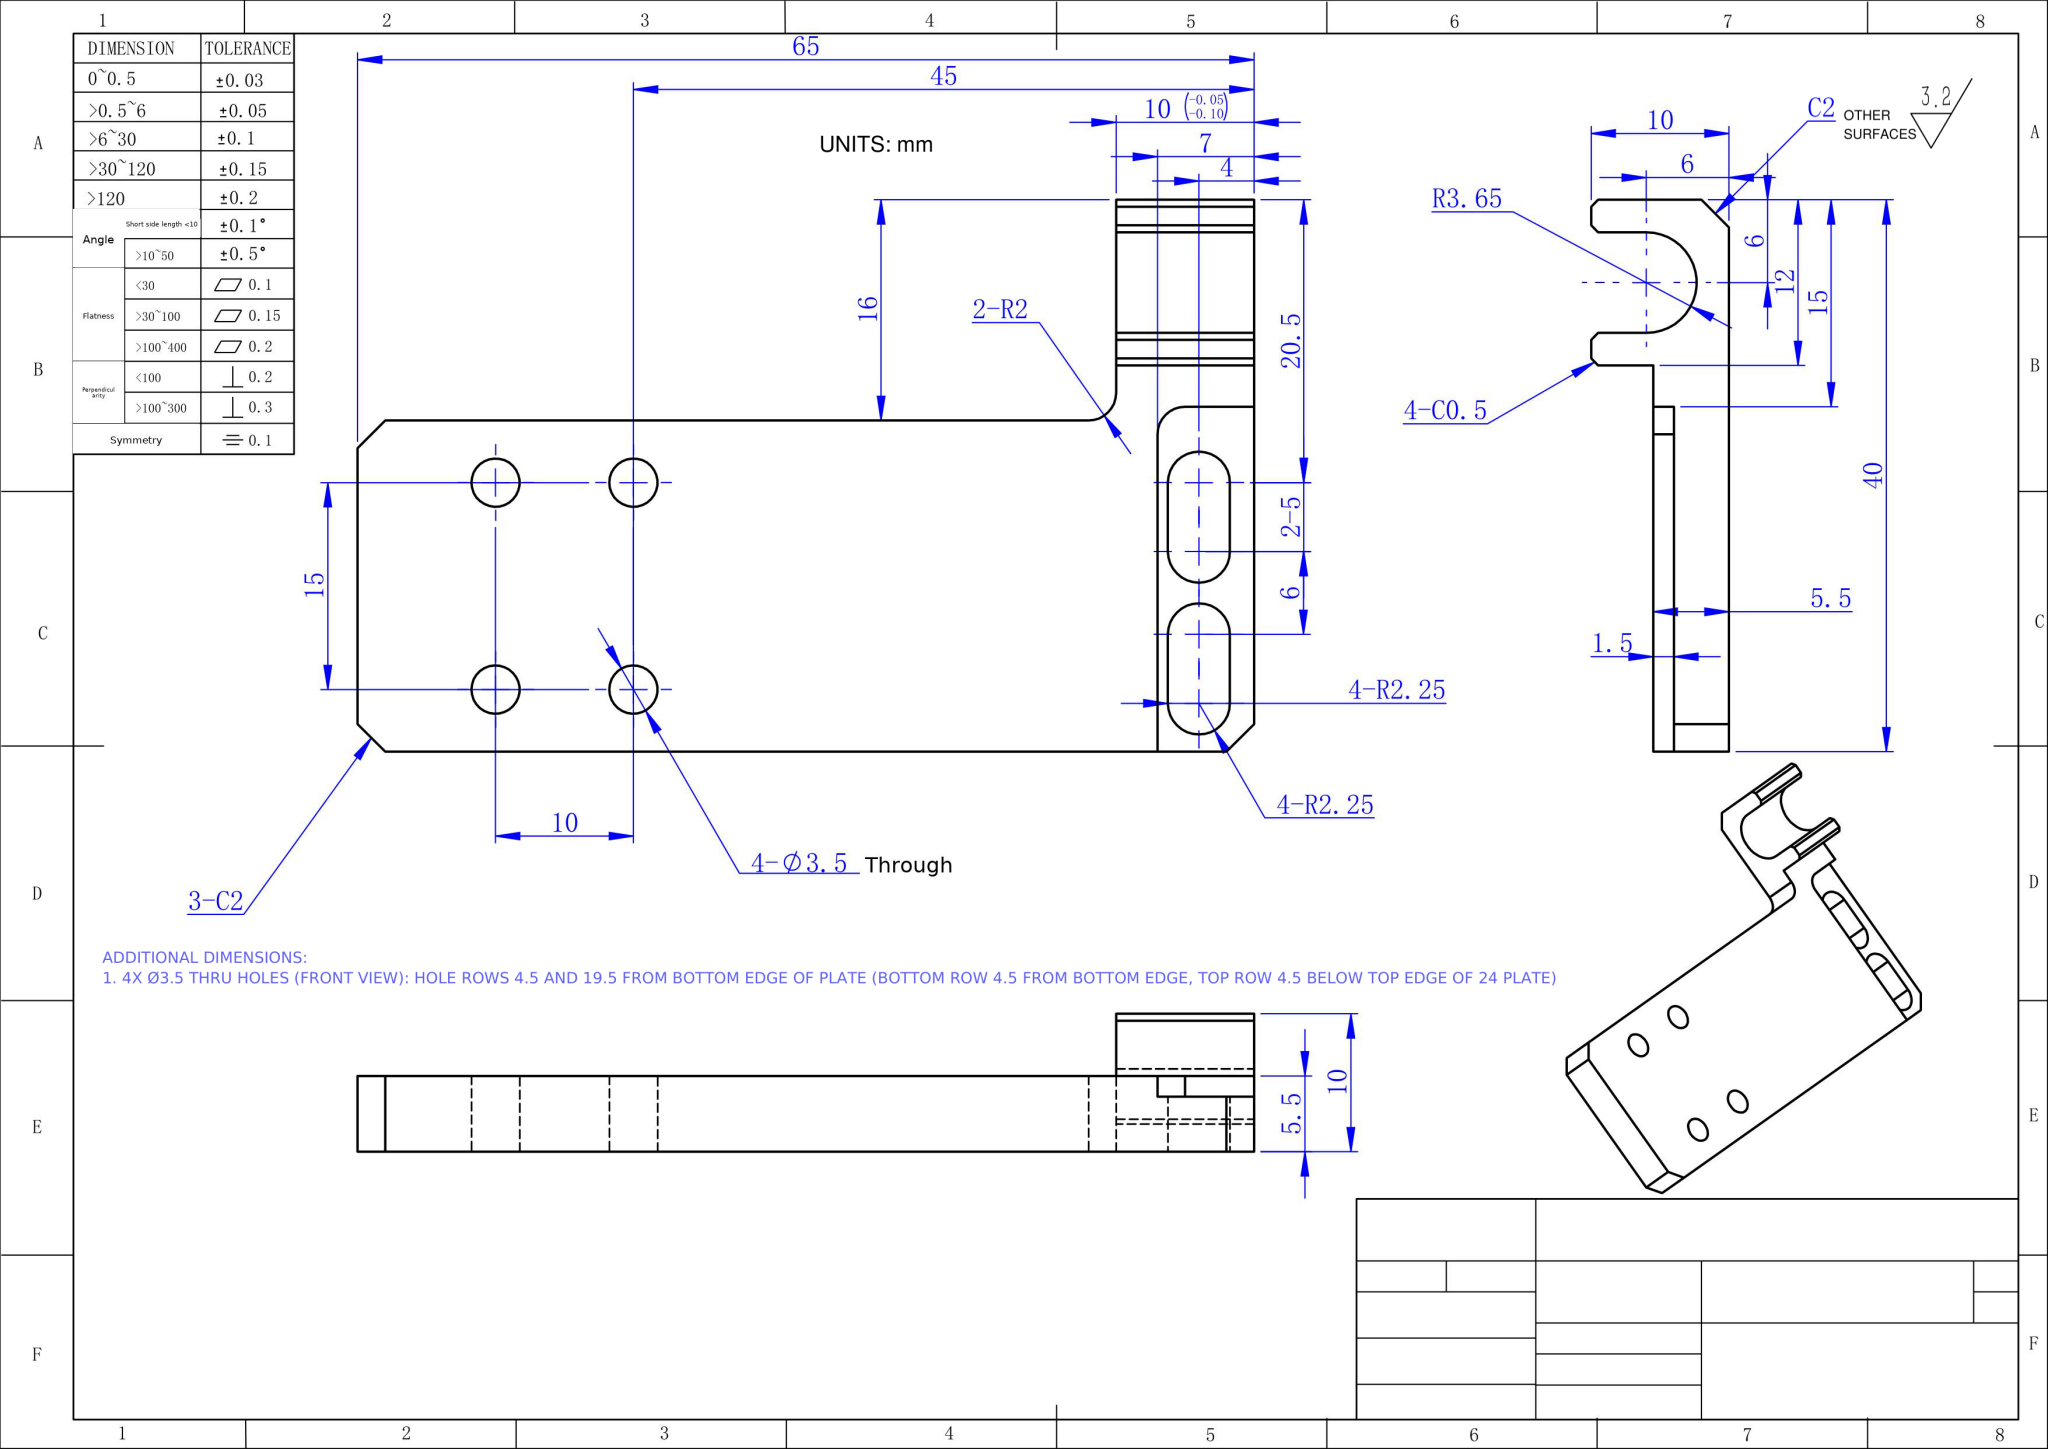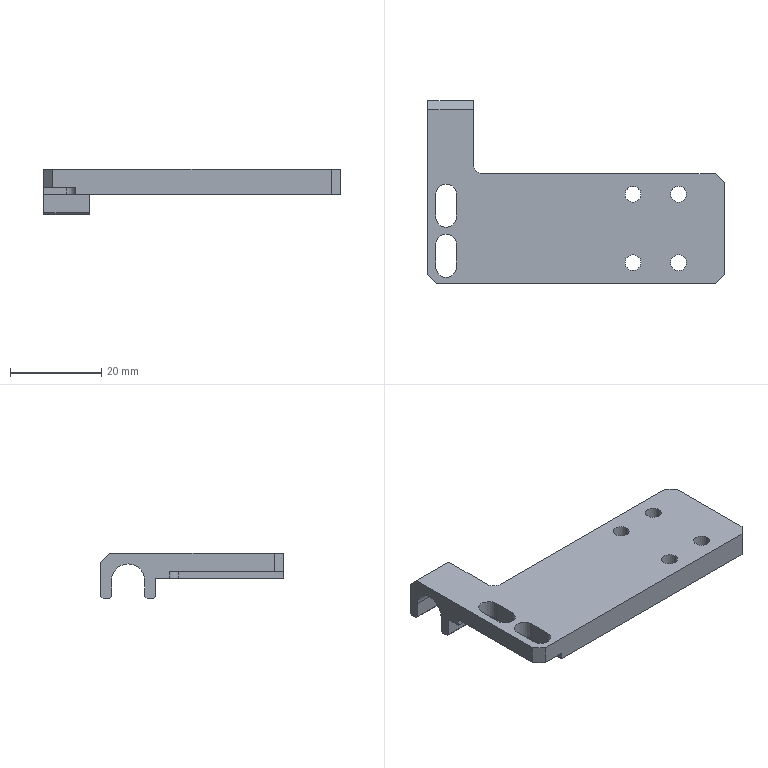Part | NX | mm | 1 solid | 44 faces | box 65 x 40 x 10 mm | volume 8668 mm3 | plane 28 | cylinder 16 | commonest cylinder face diameters 3.5 x8 4.5 x4 7.3 x2 4 x2